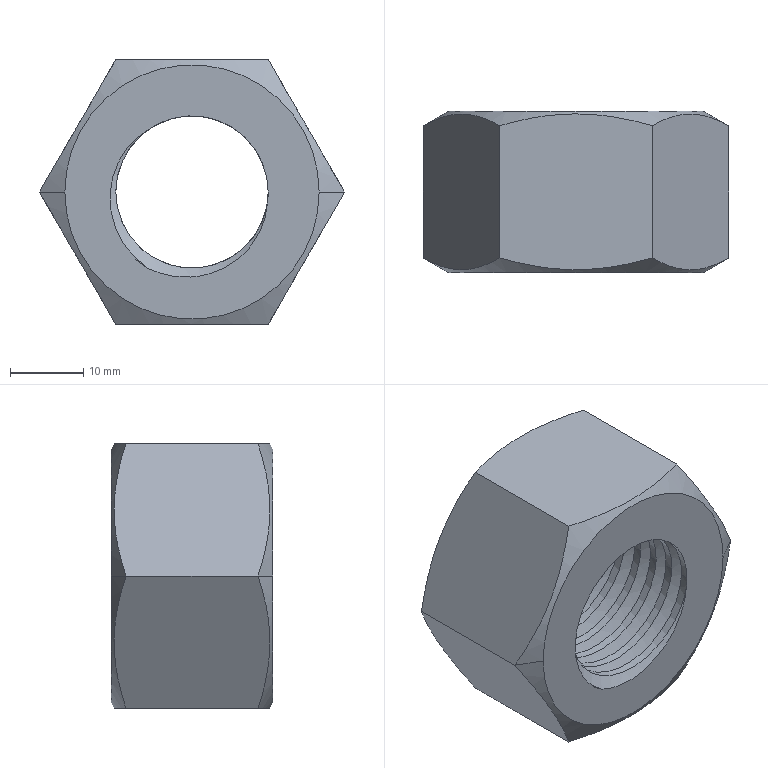Component | SolidWorks | M24-2 | 1 solid | 30 faces | volume 16274 mm3 | cylinder 16 | plane 8 | cone 4 | spline 2 | commonest cylinder face diameters 20.75 x16